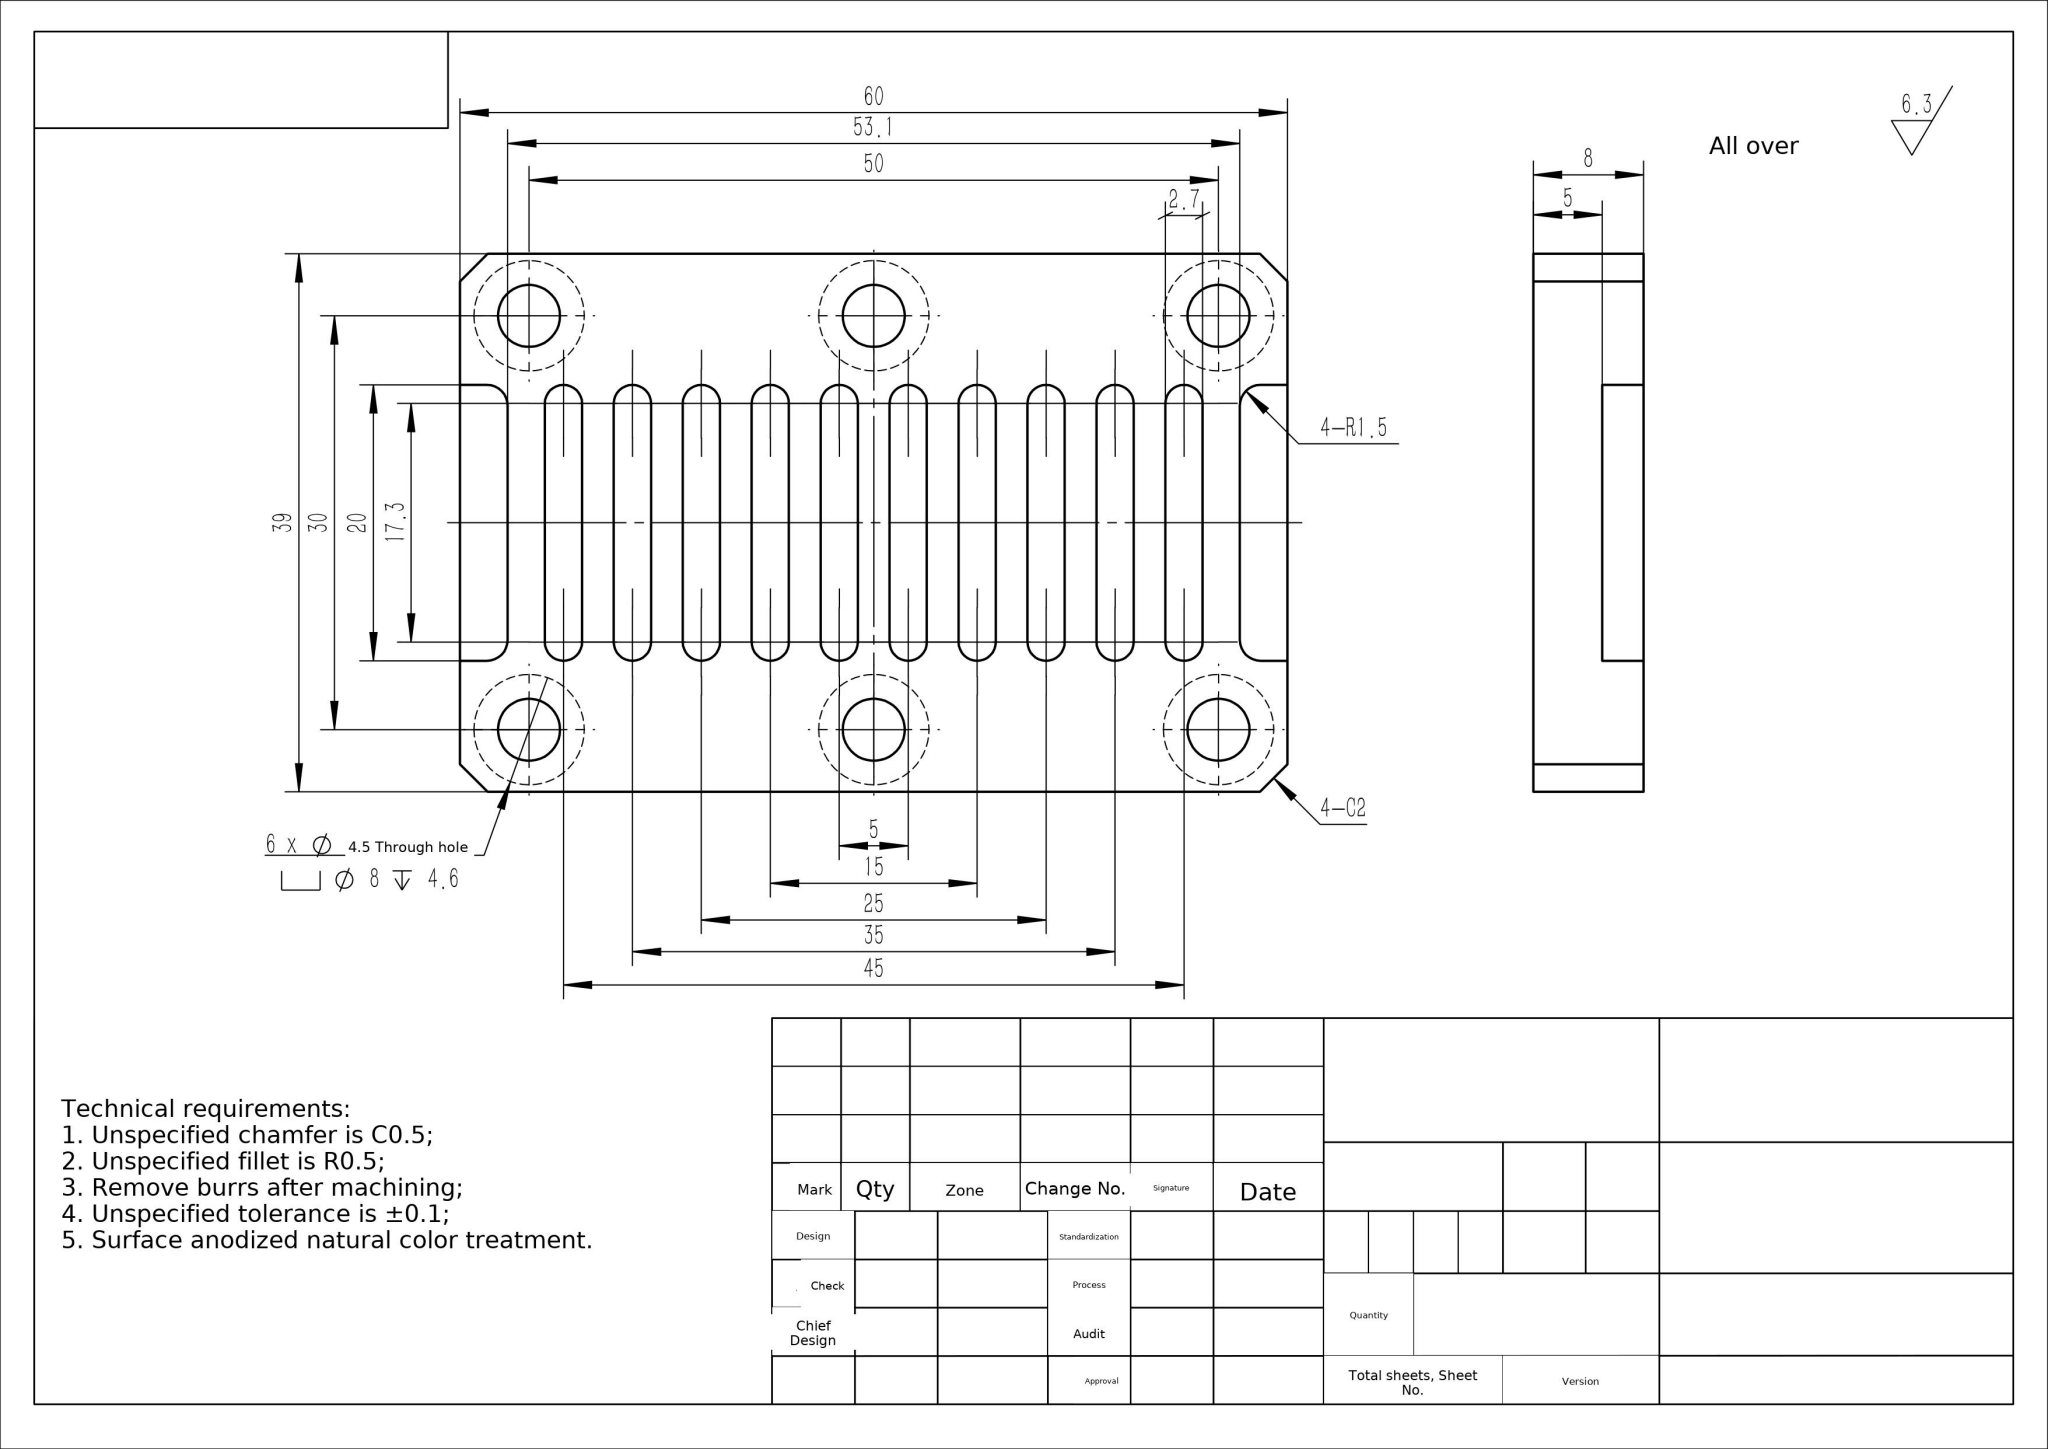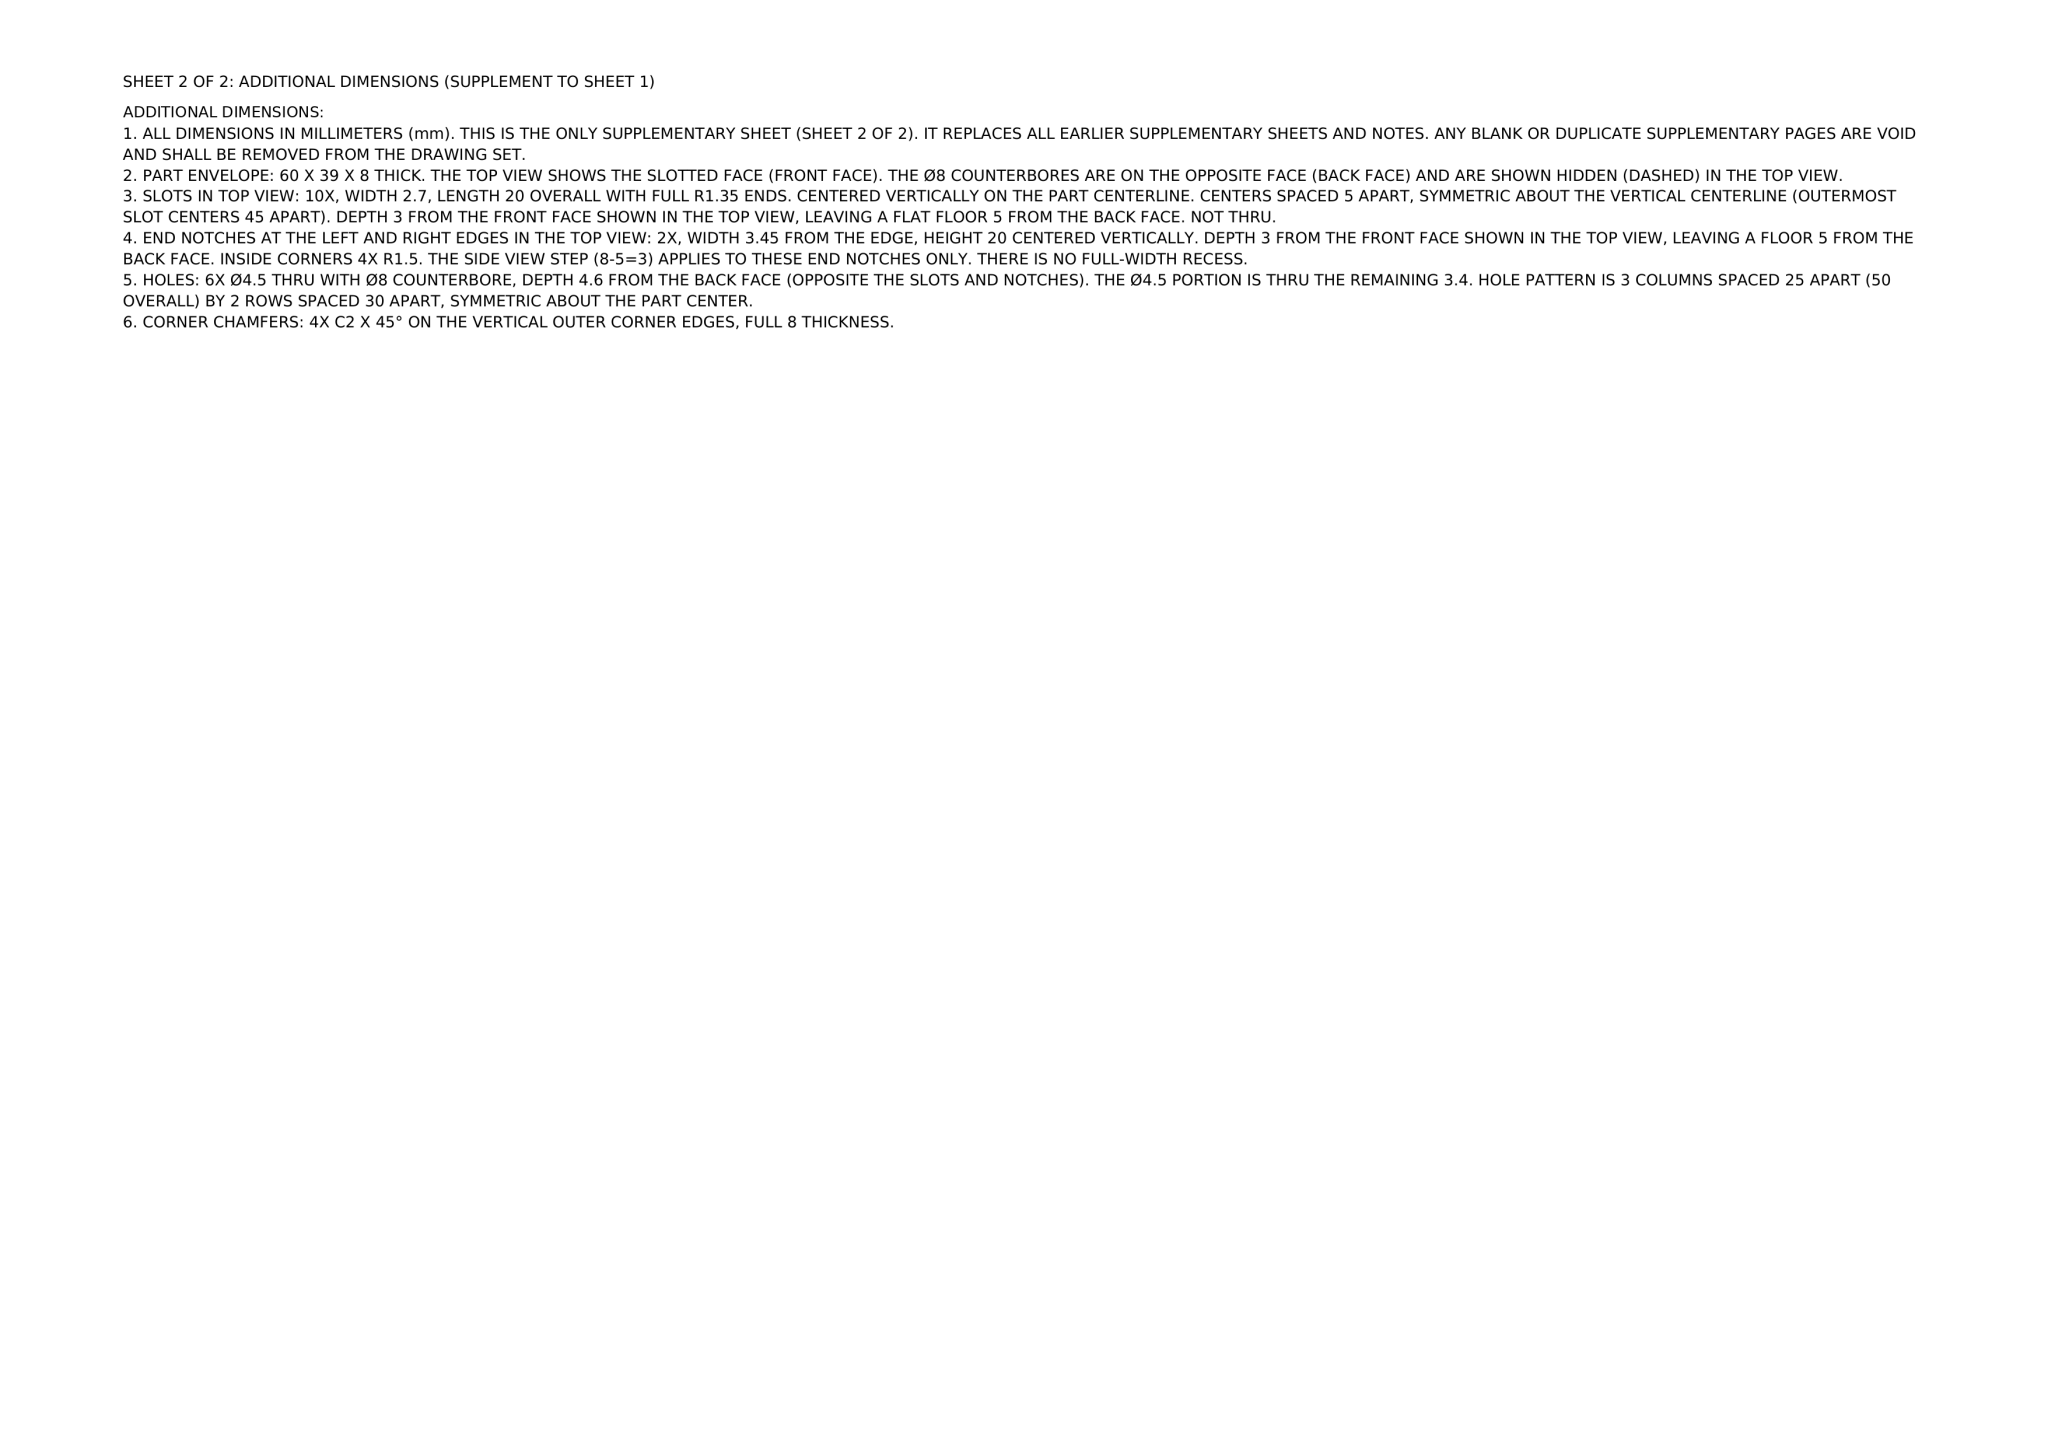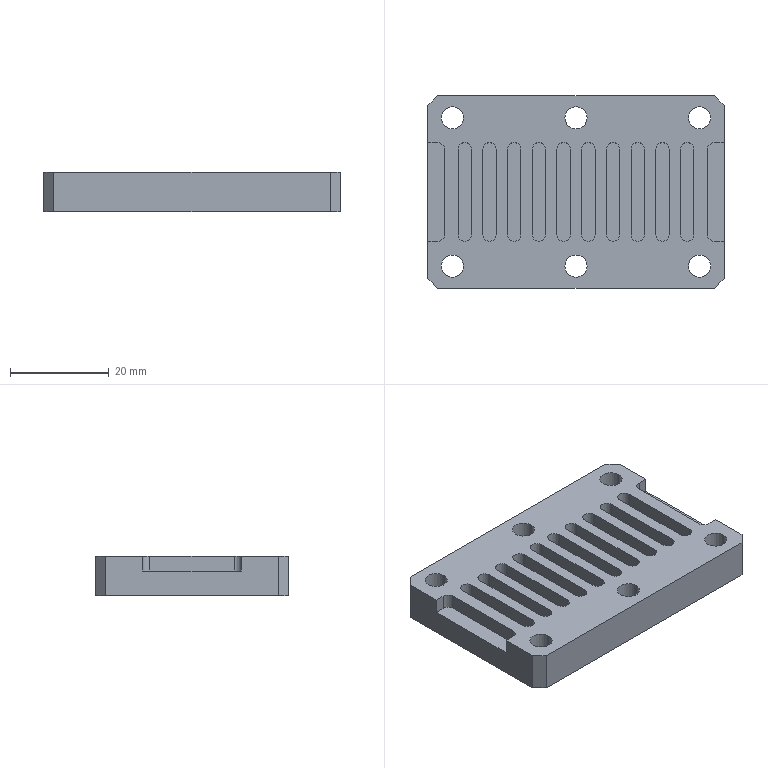Part | NX | mm | 1 solid | 102 faces | box 60 x 39 x 8 mm | volume 14963 mm3 | plane 54 | cylinder 48 | commonest cylinder face diameters 2.7 x20 8 x12 4.5 x12 3 x4